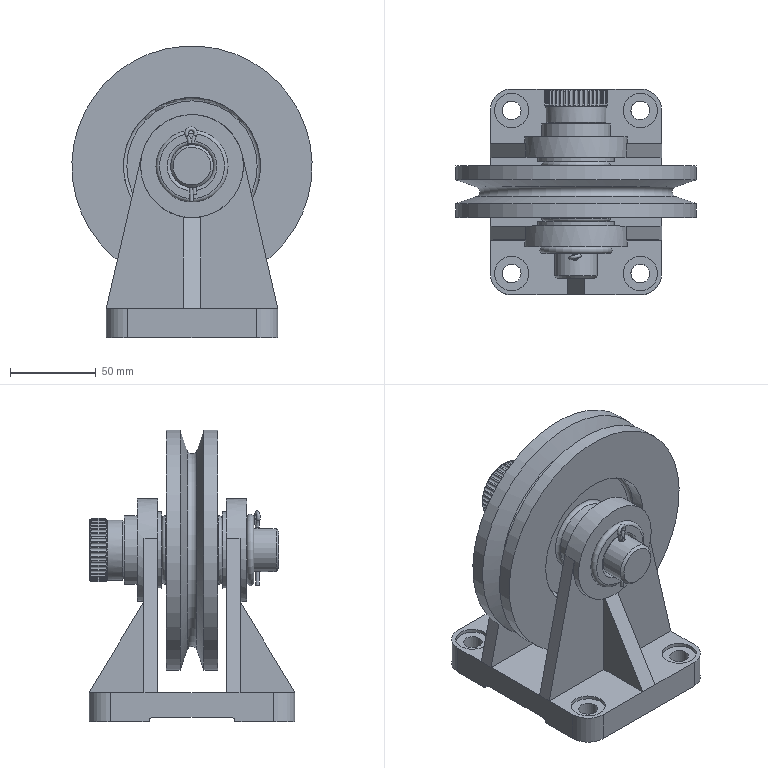Assembly | NX | mm | 7 component files | 7 solids | 296 faces | box 140 x 120 x 170 mm | volume 732455 mm3 | cylinder 129 | cone 91 | plane 64 | torus 12 | commonest cylinder face diameters 2 x42 37 x40 25 x9 5 x4 11 x4 20 x4 40 x3 4 x3
Bill of materials:
unnamed part 1 | 1 |  | Short hollow cylindrical body. About half its length has straight axial knurling or splines and the other half is a smooth cylinder of slightly smaller diameter. A central through-bore with stepped internal diameters runs through it.
unnamed part 2 | 1 |  | Hollow part, round in cross-section, with three stepped sections along its axis: a large conical (flared) head, a medium-diameter cylinder and a smaller-diameter tubular cylinder. A through-bore runs along the axis.
unnamed part 3 | 1 |  | Slender bent-wire part. A single round wire is folded back on itself to form a closed teardrop eye at one end, and the two straight legs run in parallel to free ends of different lengths.
unnamed part 4 | 1 |  | Grooved disc or wheel with a V-shaped groove around its outer rim. It has a raised central hub boss on each face, a central through-bore, and a shallow circular recess on the face around the hub.
unnamed part 5 | 1 |  | Headed cylindrical pin: a solid straight cylindrical shank with a larger flat disc head at one end and a chamfered opposite end. Two small cross-holes run through the shank.
unnamed part 6 | 1 |  | Thin flat annular ring (washer-like) with rounded or radiused edges and a large central hole.
unnamed part 7 | 1 |  | Clevis-type mounting bracket: a square base plate with rounded corners carries two parallel upright tapered lugs, each with a rounded top and an aligned through-hole. Triangular gussets brace the lugs to the base.
Mates:
1. fix | 5 1 component
2. distance | 1 1 face | 3 1 face
3. distance | 1 1 edge | 3 1 face
4. touch align | 5 1 face | 7 1 face
5. touch align | 7 1 face | 5 1 face
6. touch align | 3 1 face | 5 1 face
7. center | 4 1 face | 4 1 face | 5 1 face | 5 1 face
8. touch align | 5 1 face | 4 1 face
9. touch align | 6 1 face | 3 1 face
10. touch align | 6 1 face | 3 1 face
11. touch align | 2 1 face | 3 1 face
12. touch align | 2 1 face | 3 1 face
13. touch align | 3 1 face | 5 1 face